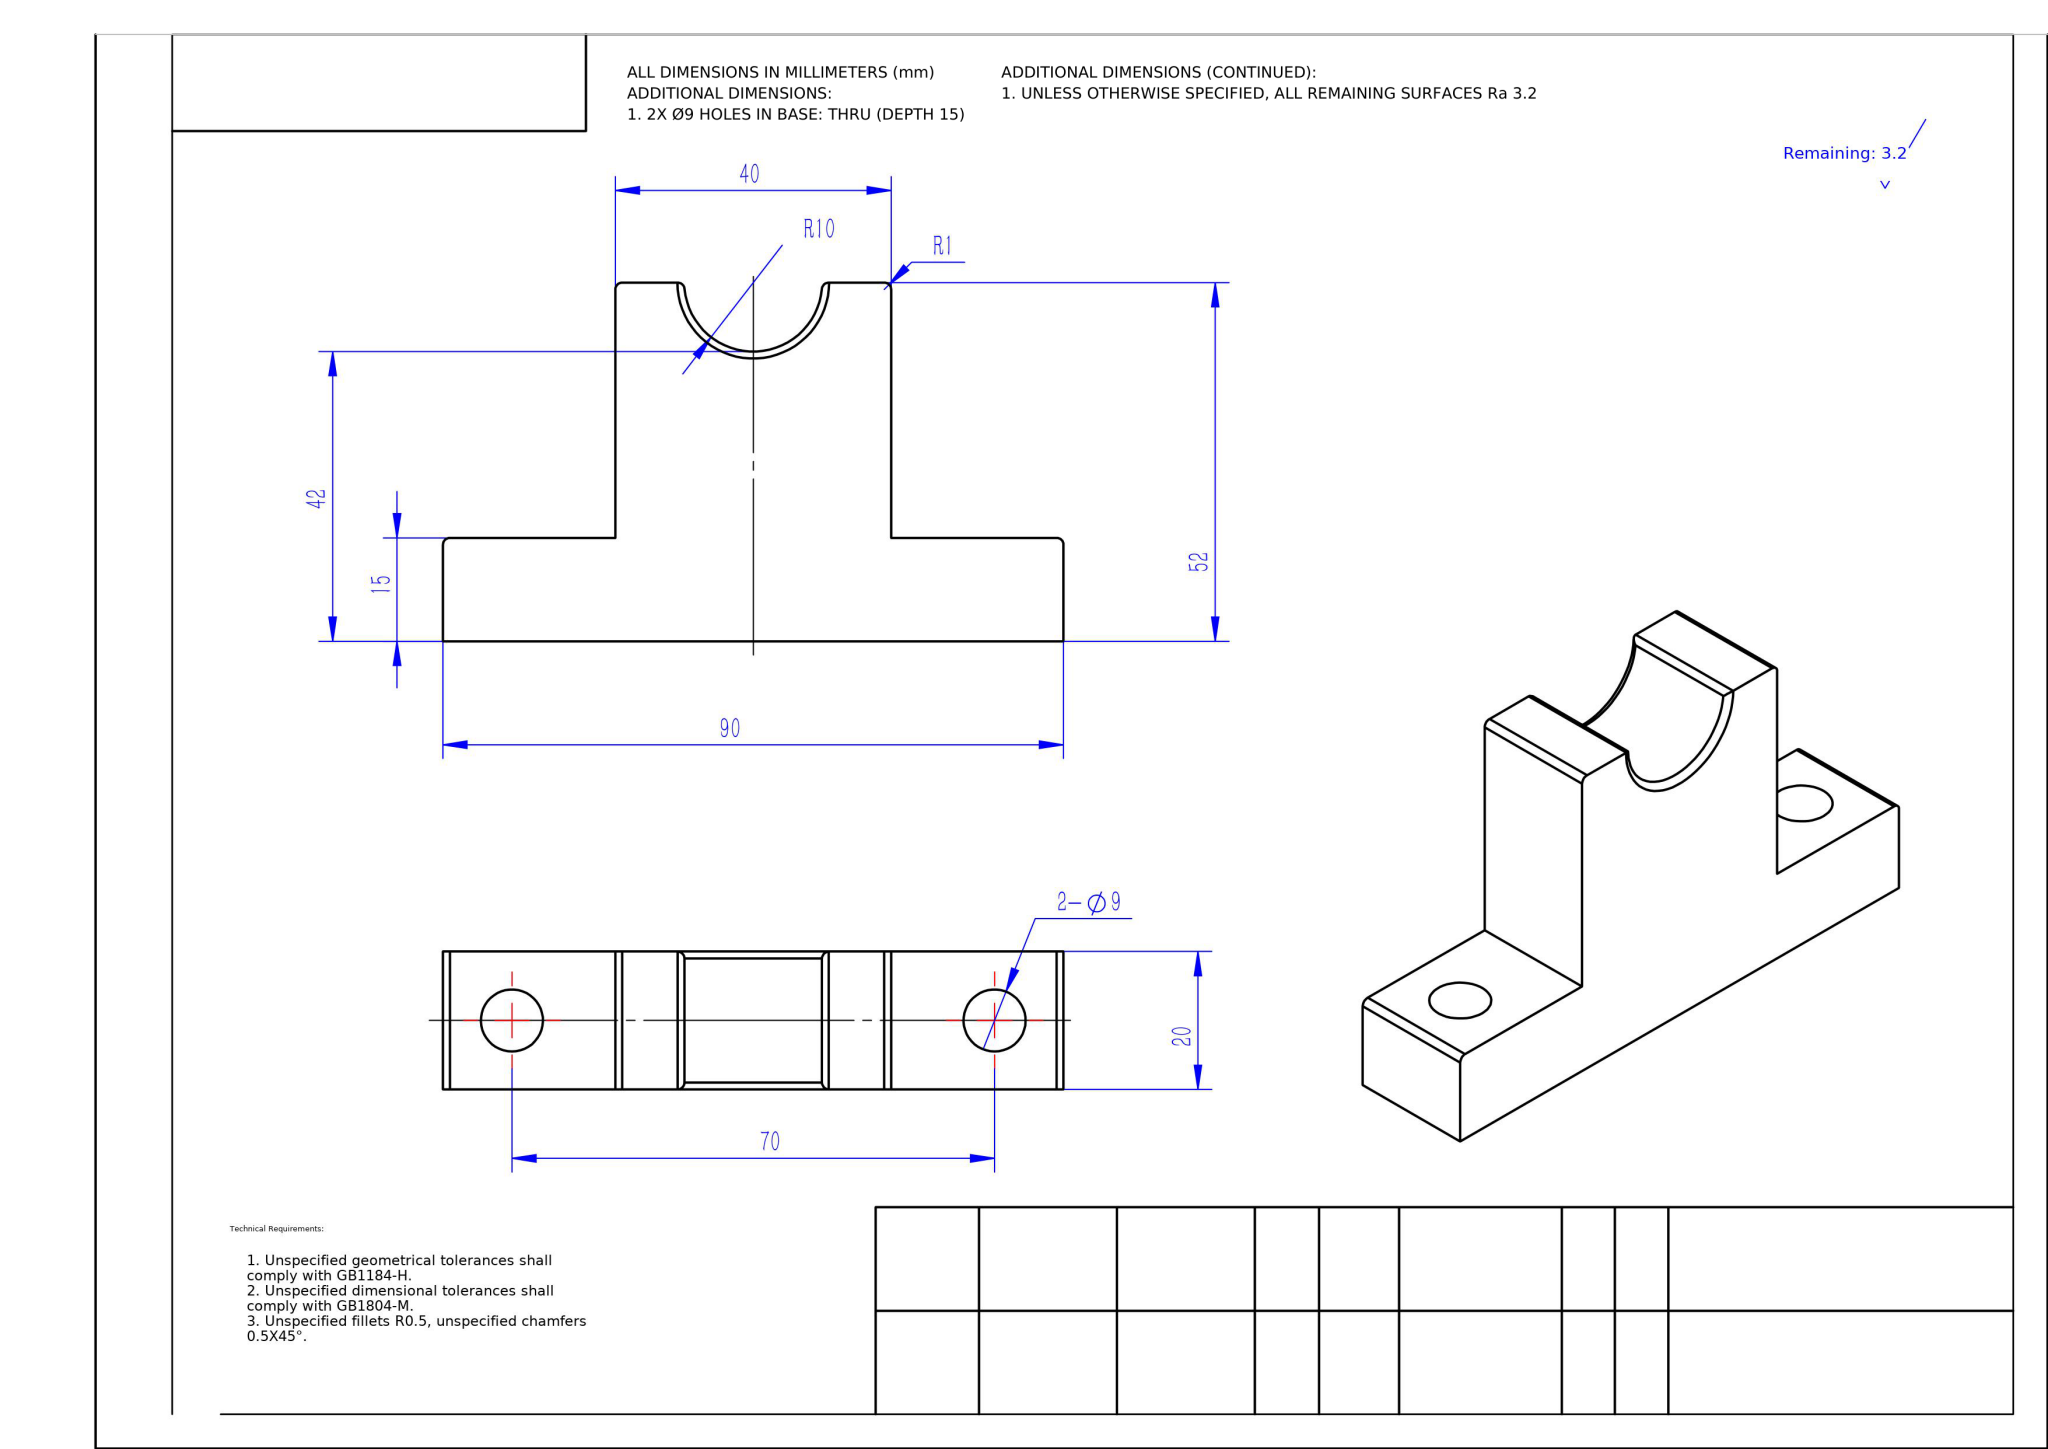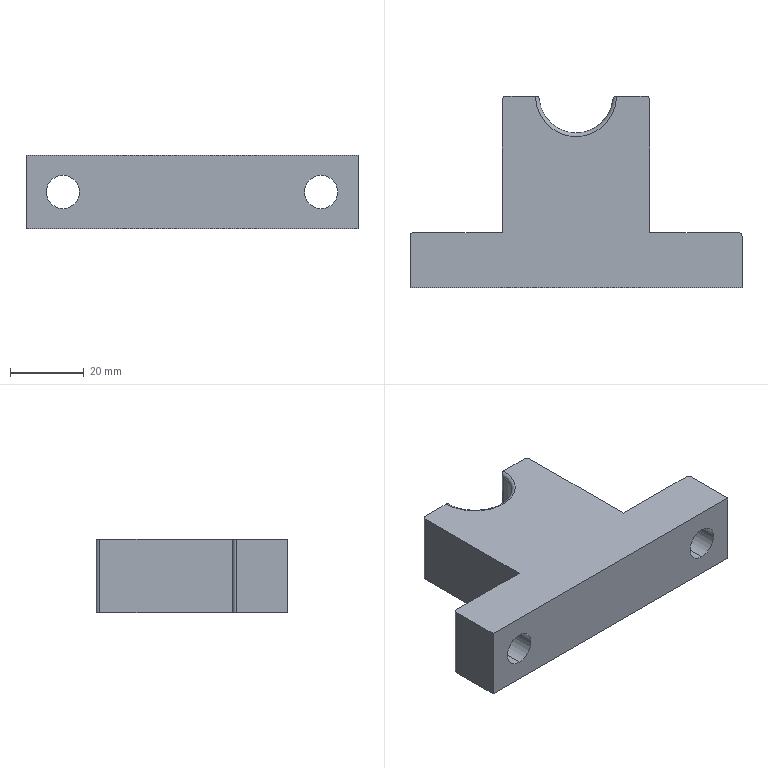Part | NX | mm | 1 solid | 24 faces | box 90 x 52 x 20 mm | volume 51512 mm3 | cylinder 11 | plane 11 | torus 2 | commonest cylinder face diameters 2 x6 9 x4 20 x1
STEP:
#1=COLOUR_RGB('',0.5294,0.549,0.549);
#2=FILL_AREA_STYLE_COLOUR('',#1);
#3=FILL_AREA_STYLE('',(#2));
#4=SURFACE_STYLE_FILL_AREA(#3);
#5=SURFACE_SIDE_STYLE('',(#4));
#6=SURFACE_STYLE_USAGE(.BOTH.,#5);
#7=PRESENTATION_STYLE_ASSIGNMENT((#6));
#8=CARTESIAN_POINT('',(-35.,0.,4.5));
#9=VERTEX_POINT('',#8);
#10=CARTESIAN_POINT('',(-35.,0.,-4.5));
#11=VERTEX_POINT('',#10);
#12=CARTESIAN_POINT('',(-35.,0.,0.));
#13=DIRECTION('',(0.,-1.,0.));
#14=DIRECTION('',(0.,0.,-1.));
#15=AXIS2_PLACEMENT_3D('',#12,#13,#14);
#16=CIRCLE('',#15,4.5);
#17=EDGE_CURVE('',#9,#11,#16,.T.);
#18=ORIENTED_EDGE('',*,*,#17,.T.);
#19=CARTESIAN_POINT('',(-35.,15.,-4.5));
#20=VERTEX_POINT('',#19);
#21=CARTESIAN_POINT('',(-35.,15.,-4.5));
#22=DIRECTION('',(0.,1.,0.));
#23=VECTOR('',#22,1000.);
#24=LINE('',#21,#23);
#25=EDGE_CURVE('',#11,#20,#24,.T.);
#26=ORIENTED_EDGE('',*,*,#25,.T.);
#27=CARTESIAN_POINT('',(-35.,15.,4.5));
#28=VERTEX_POINT('',#27);
#29=CARTESIAN_POINT('',(-35.,15.,0.));
#30=DIRECTION('',(0.,1.,0.));
#31=DIRECTION('',(0.,0.,1.));
#32=AXIS2_PLACEMENT_3D('',#29,#30,#31);
#33=CIRCLE('',#32,4.5);
#34=EDGE_CURVE('',#20,#28,#33,.T.);
#35=ORIENTED_EDGE('',*,*,#34,.T.);
#36=CARTESIAN_POINT('',(-35.,15.,4.5));
#37=DIRECTION('',(0.,1.,0.));
#38=VECTOR('',#37,1000.);
#39=LINE('',#36,#38);
#40=EDGE_CURVE('',#9,#28,#39,.T.);
#41=ORIENTED_EDGE('',*,*,#40,.F.);
#42=EDGE_LOOP('',(#18,#26,#35,#41));
#43=FACE_OUTER_BOUND('',#42,.T.);
#44=CARTESIAN_POINT('',(-35.,15.,0.));
#45=DIRECTION('',(0.,1.,0.));
#46=DIRECTION('',(0.,0.,1.));
#47=AXIS2_PLACEMENT_3D('',#44,#45,#46);
#48=CYLINDRICAL_SURFACE('',#47,4.5);
#49=ADVANCED_FACE('',(#43),#48,.F.);
#50=CARTESIAN_POINT('',(35.,0.,4.5));
#51=VERTEX_POINT('',#50);
#52=CARTESIAN_POINT('',(35.,0.,-4.5));
#53=VERTEX_POINT('',#52);
#54=CARTESIAN_POINT('',(35.,0.,0.));
#55=DIRECTION('',(0.,-1.,0.));
#56=DIRECTION('',(0.,0.,-1.));
#57=AXIS2_PLACEMENT_3D('',#54,#55,#56);
#58=CIRCLE('',#57,4.5);
#59=EDGE_CURVE('',#51,#53,#58,.T.);
#60=ORIENTED_EDGE('',*,*,#59,.T.);
#61=CARTESIAN_POINT('',(35.,15.,-4.5));
#62=VERTEX_POINT('',#61);
#63=CARTESIAN_POINT('',(35.,15.,-4.5));
#64=DIRECTION('',(0.,1.,0.));
#65=VECTOR('',#64,1000.);
#66=LINE('',#63,#65);
#67=EDGE_CURVE('',#53,#62,#66,.T.);
#68=ORIENTED_EDGE('',*,*,#67,.T.);
#69=CARTESIAN_POINT('',(35.,15.,4.5));
#70=VERTEX_POINT('',#69);
#71=CARTESIAN_POINT('',(35.,15.,0.));
#72=DIRECTION('',(0.,1.,0.));
#73=DIRECTION('',(0.,0.,1.));
#74=AXIS2_PLACEMENT_3D('',#71,#72,#73);
#75=CIRCLE('',#74,4.5);
#76=EDGE_CURVE('',#62,#70,#75,.T.);
#77=ORIENTED_EDGE('',*,*,#76,.T.);
#78=CARTESIAN_POINT('',(35.,15.,4.5));
#79=DIRECTION('',(0.,1.,0.));
#80=VECTOR('',#79,1000.);
#81=LINE('',#78,#80);
#82=EDGE_CURVE('',#51,#70,#81,.T.);
#83=ORIENTED_EDGE('',*,*,#82,.F.);
#84=EDGE_LOOP('',(#60,#68,#77,#83));
#85=FACE_OUTER_BOUND('',#84,.T.);
#86=CARTESIAN_POINT('',(35.,15.,0.));
#87=DIRECTION('',(0.,1.,0.));
#88=DIRECTION('',(0.,0.,1.));
#89=AXIS2_PLACEMENT_3D('',#86,#87,#88);
#90=CYLINDRICAL_SURFACE('',#89,4.5);
#91=ADVANCED_FACE('',(#85),#90,.F.);
#92=CARTESIAN_POINT('',(11.,52.,10.));
#93=VERTEX_POINT('',#92);
#94=CARTESIAN_POINT('',(19.,52.,10.));
#95=VERTEX_POINT('',#94);
#96=CARTESIAN_POINT('',(-45.,52.,10.));
#97=DIRECTION('',(1.,0.,0.));
#98=VECTOR('',#97,1000.);
#99=LINE('',#96,#98);
#100=EDGE_CURVE('',#93,#95,#99,.T.);
#101=ORIENTED_EDGE('',*,*,#100,.T.);
#102=CARTESIAN_POINT('',(19.,52.,-10.));
#103=VERTEX_POINT('',#102);
#104=CARTESIAN_POINT('',(19.,52.,-0.));
#105=DIRECTION('',(-0.,0.,-1.));
#106=VECTOR('',#105,1000.);
#107=LINE('',#104,#106);
#108=EDGE_CURVE('',#95,#103,#107,.T.);
#109=ORIENTED_EDGE('',*,*,#108,.T.);
#110=CARTESIAN_POINT('',(11.,52.,-10.));
#111=VERTEX_POINT('',#110);
#112=CARTESIAN_POINT('',(-45.,52.,-10.));
#113=DIRECTION('',(-1.,0.,0.));
#114=VECTOR('',#113,1000.);
#115=LINE('',#112,#114);
#116=EDGE_CURVE('',#103,#111,#115,.T.);
#117=ORIENTED_EDGE('',*,*,#116,.T.);
#118=CARTESIAN_POINT('',(10.954,52.,-9.999));
#119=VERTEX_POINT('',#118);
#120=CARTESIAN_POINT('',(11.,52.,-9.));
#121=DIRECTION('',(0.,1.,0.));
#122=DIRECTION('',(-0.,0.,-1.));
#123=AXIS2_PLACEMENT_3D('',#120,#121,#122);
#124=CIRCLE('',#123,1.);
#125=EDGE_CURVE('',#111,#119,#124,.T.);
#126=ORIENTED_EDGE('',*,*,#125,.T.);
#127=CARTESIAN_POINT('',(10.954,52.,9.999));
#128=VERTEX_POINT('',#127);
#129=CARTESIAN_POINT('',(10.954,52.,0.));
#130=DIRECTION('',(0.,0.,1.));
#131=VECTOR('',#130,1000.);
#132=LINE('',#129,#131);
#133=EDGE_CURVE('',#119,#128,#132,.T.);
#134=ORIENTED_EDGE('',*,*,#133,.T.);
#135=CARTESIAN_POINT('',(11.,52.,9.));
#136=DIRECTION('',(0.,1.,0.));
#137=DIRECTION('',(0.,0.,-1.));
#138=AXIS2_PLACEMENT_3D('',#135,#136,#137);
#139=CIRCLE('',#138,1.);
#140=EDGE_CURVE('',#128,#93,#139,.T.);
#141=ORIENTED_EDGE('',*,*,#140,.T.);
#142=EDGE_LOOP('',(#101,#109,#117,#126,#134,#141));
#143=FACE_OUTER_BOUND('',#142,.T.);
#144=CARTESIAN_POINT('',(0.,52.,0.));
#145=DIRECTION('',(0.,-1.,0.));
#146=DIRECTION('',(0.,0.,-1.));
#147=AXIS2_PLACEMENT_3D('',#144,#145,#146);
#148=PLANE('',#147);
#149=ADVANCED_FACE('',(#143),#148,.F.);
#150=CARTESIAN_POINT('',(45.,14.,-10.));
#151=VERTEX_POINT('',#150);
#152=CARTESIAN_POINT('',(45.,0.,-10.));
#153=VERTEX_POINT('',#152);
#154=CARTESIAN_POINT('',(45.,52.,-10.));
#155=DIRECTION('',(0.,-1.,0.));
#156=VECTOR('',#155,1000.);
#157=LINE('',#154,#156);
#158=EDGE_CURVE('',#151,#153,#157,.T.);
#159=ORIENTED_EDGE('',*,*,#158,.F.);
#160=CARTESIAN_POINT('',(45.,14.,10.));
#161=VERTEX_POINT('',#160);
#162=CARTESIAN_POINT('',(45.,14.,10.));
#163=DIRECTION('',(0.,0.,1.));
#164=VECTOR('',#163,1000.);
#165=LINE('',#162,#164);
#166=EDGE_CURVE('',#151,#161,#165,.T.);
#167=ORIENTED_EDGE('',*,*,#166,.T.);
#168=CARTESIAN_POINT('',(45.,0.,10.));
#169=VERTEX_POINT('',#168);
#170=CARTESIAN_POINT('',(45.,52.,10.));
#171=DIRECTION('',(0.,-1.,0.));
#172=VECTOR('',#171,1000.);
#173=LINE('',#170,#172);
#174=EDGE_CURVE('',#161,#169,#173,.T.);
#175=ORIENTED_EDGE('',*,*,#174,.T.);
#176=CARTESIAN_POINT('',(45.,0.,10.));
#177=DIRECTION('',(0.,0.,-1.));
#178=VECTOR('',#177,1000.);
#179=LINE('',#176,#178);
#180=EDGE_CURVE('',#169,#153,#179,.T.);
#181=ORIENTED_EDGE('',*,*,#180,.T.);
#182=EDGE_LOOP('',(#159,#167,#175,#181));
#183=FACE_OUTER_BOUND('',#182,.T.);
#184=CARTESIAN_POINT('',(45.,52.,10.));
#185=DIRECTION('',(-1.,0.,0.));
#186=DIRECTION('',(0.,0.,1.));
#187=AXIS2_PLACEMENT_3D('',#184,#185,#186);
#188=PLANE('',#187);
#189=ADVANCED_FACE('',(#183),#188,.F.);
#190=CARTESIAN_POINT('',(-45.,14.,10.));
#191=VERTEX_POINT('',#190);
#192=CARTESIAN_POINT('',(-45.,0.,10.));
#193=VERTEX_POINT('',#192);
#194=CARTESIAN_POINT('',(-45.,52.,10.));
#195=DIRECTION('',(0.,-1.,0.));
#196=VECTOR('',#195,1000.);
#197=LINE('',#194,#196);
#198=EDGE_CURVE('',#191,#193,#197,.T.);
#199=ORIENTED_EDGE('',*,*,#198,.F.);
#200=CARTESIAN_POINT('',(-45.,14.,-10.));
#201=VERTEX_POINT('',#200);
#202=CARTESIAN_POINT('',(-45.,14.,-10.));
#203=DIRECTION('',(0.,0.,-1.));
#204=VECTOR('',#203,1000.);
#205=LINE('',#202,#204);
#206=EDGE_CURVE('',#191,#201,#205,.T.);
#207=ORIENTED_EDGE('',*,*,#206,.T.);
#208=CARTESIAN_POINT('',(-45.,0.,-10.));
#209=VERTEX_POINT('',#208);
#210=CARTESIAN_POINT('',(-45.,52.,-10.));
#211=DIRECTION('',(0.,-1.,0.));
#212=VECTOR('',#211,1000.);
#213=LINE('',#210,#212);
#214=EDGE_CURVE('',#201,#209,#213,.T.);
#215=ORIENTED_EDGE('',*,*,#214,.T.);
#216=CARTESIAN_POINT('',(-45.,0.,10.));
#217=DIRECTION('',(0.,0.,1.));
#218=VECTOR('',#217,1000.);
#219=LINE('',#216,#218);
#220=EDGE_CURVE('',#209,#193,#219,.T.);
#221=ORIENTED_EDGE('',*,*,#220,.T.);
#222=EDGE_LOOP('',(#199,#207,#215,#221));
#223=FACE_OUTER_BOUND('',#222,.T.);
#224=CARTESIAN_POINT('',(-45.,52.,10.));
#225=DIRECTION('',(1.,0.,0.));
#226=DIRECTION('',(0.,0.,-1.));
#227=AXIS2_PLACEMENT_3D('',#224,#225,#226);
#228=PLANE('',#227);
#229=ADVANCED_FACE('',(#223),#228,.F.);
#230=CARTESIAN_POINT('',(-11.,52.,-10.));
#231=VERTEX_POINT('',#230);
#232=CARTESIAN_POINT('',(-19.,52.,-10.));
#233=VERTEX_POINT('',#232);
#234=CARTESIAN_POINT('',(-45.,52.,-10.));
#235=DIRECTION('',(-1.,0.,0.));
#236=VECTOR('',#235,1000.);
#237=LINE('',#234,#236);
#238=EDGE_CURVE('',#231,#233,#237,.T.);
#239=ORIENTED_EDGE('',*,*,#238,.F.);
#240=CARTESIAN_POINT('',(0.,52.,-10.));
#241=DIRECTION('',(0.,0.,1.));
#242=DIRECTION('',(1.,0.,0.));
#243=AXIS2_PLACEMENT_3D('',#240,#241,#242);
#244=CIRCLE('',#243,11.);
#245=EDGE_CURVE('',#231,#111,#244,.T.);
#246=ORIENTED_EDGE('',*,*,#245,.T.);
#247=ORIENTED_EDGE('',*,*,#116,.F.);
#248=CARTESIAN_POINT('',(20.,51.,-10.));
#249=VERTEX_POINT('',#248);
#250=CARTESIAN_POINT('',(19.,51.,-10.));
#251=DIRECTION('',(0.,0.,-1.));
#252=DIRECTION('',(1.,0.,0.));
#253=AXIS2_PLACEMENT_3D('',#250,#251,#252);
#254=CIRCLE('',#253,1.);
#255=EDGE_CURVE('',#103,#249,#254,.T.);
#256=ORIENTED_EDGE('',*,*,#255,.T.);
#257=CARTESIAN_POINT('',(20.,15.,-10.));
#258=VERTEX_POINT('',#257);
#259=CARTESIAN_POINT('',(20.,15.,-10.));
#260=DIRECTION('',(0.,1.,0.));
#261=VECTOR('',#260,1000.);
#262=LINE('',#259,#261);
#263=EDGE_CURVE('',#258,#249,#262,.T.);
#264=ORIENTED_EDGE('',*,*,#263,.F.);
#265=CARTESIAN_POINT('',(44.,15.,-10.));
#266=VERTEX_POINT('',#265);
#267=CARTESIAN_POINT('',(20.,15.,-10.));
#268=DIRECTION('',(-1.,0.,0.));
#269=VECTOR('',#268,1000.);
#270=LINE('',#267,#269);
#271=EDGE_CURVE('',#266,#258,#270,.T.);
#272=ORIENTED_EDGE('',*,*,#271,.F.);
#273=CARTESIAN_POINT('',(44.,14.,-10.));
#274=DIRECTION('',(0.,0.,-1.));
#275=DIRECTION('',(1.,-0.,0.));
#276=AXIS2_PLACEMENT_3D('',#273,#274,#275);
#277=CIRCLE('',#276,1.);
#278=EDGE_CURVE('',#266,#151,#277,.T.);
#279=ORIENTED_EDGE('',*,*,#278,.T.);
#280=ORIENTED_EDGE('',*,*,#158,.T.);
#281=CARTESIAN_POINT('',(-45.,0.,-10.));
#282=DIRECTION('',(-1.,0.,0.));
#283=VECTOR('',#282,1000.);
#284=LINE('',#281,#283);
#285=EDGE_CURVE('',#153,#209,#284,.T.);
#286=ORIENTED_EDGE('',*,*,#285,.T.);
#287=ORIENTED_EDGE('',*,*,#214,.F.);
#288=CARTESIAN_POINT('',(-44.,15.,-10.));
#289=VERTEX_POINT('',#288);
#290=CARTESIAN_POINT('',(-44.,14.,-10.));
#291=DIRECTION('',(0.,0.,-1.));
#292=DIRECTION('',(1.,0.,0.));
#293=AXIS2_PLACEMENT_3D('',#290,#291,#292);
#294=CIRCLE('',#293,1.);
#295=EDGE_CURVE('',#201,#289,#294,.T.);
#296=ORIENTED_EDGE('',*,*,#295,.T.);
#297=CARTESIAN_POINT('',(-20.,15.,-10.));
#298=VERTEX_POINT('',#297);
#299=CARTESIAN_POINT('',(-45.,15.,-10.));
#300=DIRECTION('',(-1.,0.,0.));
#301=VECTOR('',#300,1000.);
#302=LINE('',#299,#301);
#303=EDGE_CURVE('',#298,#289,#302,.T.);
#304=ORIENTED_EDGE('',*,*,#303,.F.);
#305=CARTESIAN_POINT('',(-20.,51.,-10.));
#306=VERTEX_POINT('',#305);
#307=CARTESIAN_POINT('',(-20.,15.,-10.));
#308=DIRECTION('',(0.,1.,0.));
#309=VECTOR('',#308,1000.);
#310=LINE('',#307,#309);
#311=EDGE_CURVE('',#298,#306,#310,.T.);
#312=ORIENTED_EDGE('',*,*,#311,.T.);
#313=CARTESIAN_POINT('',(-19.,51.,-10.));
#314=DIRECTION('',(0.,0.,-1.));
#315=DIRECTION('',(1.,0.,0.));
#316=AXIS2_PLACEMENT_3D('',#313,#314,#315);
#317=CIRCLE('',#316,1.);
#318=EDGE_CURVE('',#306,#233,#317,.T.);
#319=ORIENTED_EDGE('',*,*,#318,.T.);
#320=EDGE_LOOP('',(#239,#246,#247,#256,#264,#272,#279,#280,#286,#287,#296,#304,#312,#319));
#321=FACE_OUTER_BOUND('',#320,.T.);
#322=CARTESIAN_POINT('',(-45.,52.,-10.));
#323=DIRECTION('',(0.,0.,1.));
#324=DIRECTION('',(1.,0.,0.));
#325=AXIS2_PLACEMENT_3D('',#322,#323,#324);
#326=PLANE('',#325);
#327=ADVANCED_FACE('',(#321),#326,.F.);
#328=ORIENTED_EDGE('',*,*,#100,.F.);
#329=CARTESIAN_POINT('',(-11.,52.,10.));
#330=VERTEX_POINT('',#329);
#331=CARTESIAN_POINT('',(0.,52.,10.));
#332=DIRECTION('',(0.,0.,-1.));
#333=DIRECTION('',(-1.,0.,0.));
#334=AXIS2_PLACEMENT_3D('',#331,#332,#333);
#335=CIRCLE('',#334,11.);
#336=EDGE_CURVE('',#93,#330,#335,.T.);
#337=ORIENTED_EDGE('',*,*,#336,.T.);
#338=CARTESIAN_POINT('',(-19.,52.,10.));
#339=VERTEX_POINT('',#338);
#340=CARTESIAN_POINT('',(-45.,52.,10.));
#341=DIRECTION('',(1.,0.,0.));
#342=VECTOR('',#341,1000.);
#343=LINE('',#340,#342);
#344=EDGE_CURVE('',#339,#330,#343,.T.);
#345=ORIENTED_EDGE('',*,*,#344,.F.);
#346=CARTESIAN_POINT('',(-20.,51.,10.));
#347=VERTEX_POINT('',#346);
#348=CARTESIAN_POINT('',(-19.,51.,10.));
#349=DIRECTION('',(0.,0.,1.));
#350=DIRECTION('',(-1.,0.,0.));
#351=AXIS2_PLACEMENT_3D('',#348,#349,#350);
#352=CIRCLE('',#351,1.);
#353=EDGE_CURVE('',#339,#347,#352,.T.);
#354=ORIENTED_EDGE('',*,*,#353,.T.);
#355=CARTESIAN_POINT('',(-20.,15.,10.));
#356=VERTEX_POINT('',#355);
#357=CARTESIAN_POINT('',(-20.,15.,10.));
#358=DIRECTION('',(0.,1.,0.));
#359=VECTOR('',#358,1000.);
#360=LINE('',#357,#359);
#361=EDGE_CURVE('',#356,#347,#360,.T.);
#362=ORIENTED_EDGE('',*,*,#361,.F.);
#363=CARTESIAN_POINT('',(-44.,15.,10.));
#364=VERTEX_POINT('',#363);
#365=CARTESIAN_POINT('',(-45.,15.,10.));
#366=DIRECTION('',(1.,0.,0.));
#367=VECTOR('',#366,1000.);
#368=LINE('',#365,#367);
#369=EDGE_CURVE('',#364,#356,#368,.T.);
#370=ORIENTED_EDGE('',*,*,#369,.F.);
#371=CARTESIAN_POINT('',(-44.,14.,10.));
#372=DIRECTION('',(0.,0.,1.));
#373=DIRECTION('',(-1.,-0.,0.));
#374=AXIS2_PLACEMENT_3D('',#371,#372,#373);
#375=CIRCLE('',#374,1.);
#376=EDGE_CURVE('',#364,#191,#375,.T.);
#377=ORIENTED_EDGE('',*,*,#376,.T.);
#378=ORIENTED_EDGE('',*,*,#198,.T.);
#379=CARTESIAN_POINT('',(-45.,0.,10.));
#380=DIRECTION('',(1.,0.,0.));
#381=VECTOR('',#380,1000.);
#382=LINE('',#379,#381);
#383=EDGE_CURVE('',#193,#169,#382,.T.);
#384=ORIENTED_EDGE('',*,*,#383,.T.);
#385=ORIENTED_EDGE('',*,*,#174,.F.);
#386=CARTESIAN_POINT('',(44.,15.,10.));
#387=VERTEX_POINT('',#386);
#388=CARTESIAN_POINT('',(44.,14.,10.));
#389=DIRECTION('',(0.,0.,1.));
#390=DIRECTION('',(-1.,0.,0.));
#391=AXIS2_PLACEMENT_3D('',#388,#389,#390);
#392=CIRCLE('',#391,1.);
#393=EDGE_CURVE('',#161,#387,#392,.T.);
#394=ORIENTED_EDGE('',*,*,#393,.T.);
#395=CARTESIAN_POINT('',(20.,15.,10.));
#396=VERTEX_POINT('',#395);
#397=CARTESIAN_POINT('',(20.,15.,10.));
#398=DIRECTION('',(1.,0.,0.));
#399=VECTOR('',#398,1000.);
#400=LINE('',#397,#399);
#401=EDGE_CURVE('',#396,#387,#400,.T.);
#402=ORIENTED_EDGE('',*,*,#401,.F.);
#403=CARTESIAN_POINT('',(20.,51.,10.));
#404=VERTEX_POINT('',#403);
#405=CARTESIAN_POINT('',(20.,15.,10.));
#406=DIRECTION('',(0.,1.,0.));
#407=VECTOR('',#406,1000.);
#408=LINE('',#405,#407);
#409=EDGE_CURVE('',#396,#404,#408,.T.);
#410=ORIENTED_EDGE('',*,*,#409,.T.);
#411=CARTESIAN_POINT('',(19.,51.,10.));
#412=DIRECTION('',(0.,0.,1.));
#413=DIRECTION('',(-1.,0.,0.));
#414=AXIS2_PLACEMENT_3D('',#411,#412,#413);
#415=CIRCLE('',#414,1.);
#416=EDGE_CURVE('',#404,#95,#415,.T.);
#417=ORIENTED_EDGE('',*,*,#416,.T.);
#418=EDGE_LOOP('',(#328,#337,#345,#354,#362,#370,#377,#378,#384,#385,#394,#402,#410,#417));
#419=FACE_OUTER_BOUND('',#418,.T.);
#420=CARTESIAN_POINT('',(-45.,52.,10.));
#421=DIRECTION('',(0.,0.,-1.));
#422=DIRECTION('',(-1.,0.,0.));
#423=AXIS2_PLACEMENT_3D('',#420,#421,#422);
#424=PLANE('',#423);
#425=ADVANCED_FACE('',(#419),#424,.F.);
#426=ORIENTED_EDGE('',*,*,#238,.T.);
#427=CARTESIAN_POINT('',(-19.,52.,0.));
#428=DIRECTION('',(0.,0.,1.));
#429=VECTOR('',#428,1000.);
#430=LINE('',#427,#429);
#431=EDGE_CURVE('',#233,#339,#430,.T.);
#432=ORIENTED_EDGE('',*,*,#431,.T.);
#433=ORIENTED_EDGE('',*,*,#344,.T.);
#434=CARTESIAN_POINT('',(-10.954,52.,9.999));
#435=VERTEX_POINT('',#434);
#436=CARTESIAN_POINT('',(-11.,52.,9.));
#437=DIRECTION('',(0.,1.,0.));
#438=DIRECTION('',(0.,0.,-1.));
#439=AXIS2_PLACEMENT_3D('',#436,#437,#438);
#440=CIRCLE('',#439,1.);
#441=EDGE_CURVE('',#330,#435,#440,.T.);
#442=ORIENTED_EDGE('',*,*,#441,.T.);
#443=CARTESIAN_POINT('',(-10.954,52.,-9.999));
#444=VERTEX_POINT('',#443);
#445=CARTESIAN_POINT('',(-10.954,52.,0.));
#446=DIRECTION('',(0.,0.,-1.));
#447=VECTOR('',#446,1000.);
#448=LINE('',#445,#447);
#449=EDGE_CURVE('',#435,#444,#448,.T.);
#450=ORIENTED_EDGE('',*,*,#449,.T.);
#451=CARTESIAN_POINT('',(-11.,52.,-9.));
#452=DIRECTION('',(0.,1.,0.));
#453=DIRECTION('',(0.,0.,-1.));
#454=AXIS2_PLACEMENT_3D('',#451,#452,#453);
#455=CIRCLE('',#454,1.);
#456=EDGE_CURVE('',#444,#231,#455,.T.);
#457=ORIENTED_EDGE('',*,*,#456,.T.);
#458=EDGE_LOOP('',(#426,#432,#433,#442,#450,#457));
#459=FACE_OUTER_BOUND('',#458,.T.);
#460=CARTESIAN_POINT('',(0.,52.,0.));
#461=DIRECTION('',(0.,-1.,0.));
#462=DIRECTION('',(0.,0.,-1.));
#463=AXIS2_PLACEMENT_3D('',#460,#461,#462);
#464=PLANE('',#463);
#465=ADVANCED_FACE('',(#459),#464,.F.);
#466=ORIENTED_EDGE('',*,*,#17,.F.);
#467=CARTESIAN_POINT('',(-35.,0.,0.));
#468=DIRECTION('',(0.,-1.,0.));
#469=DIRECTION('',(0.,0.,-1.));
#470=AXIS2_PLACEMENT_3D('',#467,#468,#469);
#471=CIRCLE('',#470,4.5);
#472=EDGE_CURVE('',#11,#9,#471,.T.);
#473=ORIENTED_EDGE('',*,*,#472,.F.);
#474=EDGE_LOOP('',(#466,#473));
#475=FACE_BOUND('',#474,.T.);
#476=ORIENTED_EDGE('',*,*,#59,.F.);
#477=CARTESIAN_POINT('',(35.,0.,0.));
#478=DIRECTION('',(0.,-1.,0.));
#479=DIRECTION('',(0.,0.,-1.));
#480=AXIS2_PLACEMENT_3D('',#477,#478,#479);
#481=CIRCLE('',#480,4.5);
#482=EDGE_CURVE('',#53,#51,#481,.T.);
#483=ORIENTED_EDGE('',*,*,#482,.F.);
#484=EDGE_LOOP('',(#476,#483));
#485=FACE_BOUND('',#484,.T.);
#486=ORIENTED_EDGE('',*,*,#180,.F.);
#487=ORIENTED_EDGE('',*,*,#383,.F.);
#488=ORIENTED_EDGE('',*,*,#220,.F.);
#489=ORIENTED_EDGE('',*,*,#285,.F.);
#490=EDGE_LOOP('',(#486,#487,#488,#489));
#491=FACE_OUTER_BOUND('',#490,.T.);
#492=CARTESIAN_POINT('',(0.,0.,0.));
#493=DIRECTION('',(0.,-1.,0.));
#494=DIRECTION('',(0.,0.,-1.));
#495=AXIS2_PLACEMENT_3D('',#492,#493,#494);
#496=PLANE('',#495);
#497=ADVANCED_FACE('',(#475,#485,#491),#496,.T.);
#498=ORIENTED_EDGE('',*,*,#263,.T.);
#499=CARTESIAN_POINT('',(20.,51.,-10.));
#500=DIRECTION('',(0.,0.,1.));
#501=VECTOR('',#500,1000.);
#502=LINE('',#499,#501);
#503=EDGE_CURVE('',#249,#404,#502,.T.);
#504=ORIENTED_EDGE('',*,*,#503,.T.);
#505=ORIENTED_EDGE('',*,*,#409,.F.);
#506=CARTESIAN_POINT('',(20.,15.,-10.));
#507=DIRECTION('',(0.,0.,1.));
#508=VECTOR('',#507,1000.);
#509=LINE('',#506,#508);
#510=EDGE_CURVE('',#258,#396,#509,.T.);
#511=ORIENTED_EDGE('',*,*,#510,.F.);
#512=EDGE_LOOP('',(#498,#504,#505,#511));
#513=FACE_OUTER_BOUND('',#512,.T.);
#514=CARTESIAN_POINT('',(20.,15.,-10.));
#515=DIRECTION('',(-1.,0.,0.));
#516=DIRECTION('',(0.,0.,1.));
#517=AXIS2_PLACEMENT_3D('',#514,#515,#516);
#518=PLANE('',#517);
#519=ADVANCED_FACE('',(#513),#518,.F.);
#520=CARTESIAN_POINT('',(35.,15.,0.));
#521=DIRECTION('',(0.,1.,0.));
#522=DIRECTION('',(0.,0.,1.));
#523=AXIS2_PLACEMENT_3D('',#520,#521,#522);
#524=CIRCLE('',#523,4.5);
#525=EDGE_CURVE('',#70,#62,#524,.T.);
#526=ORIENTED_EDGE('',*,*,#525,.F.);
#527=ORIENTED_EDGE('',*,*,#76,.F.);
#528=EDGE_LOOP('',(#526,#527));
#529=FACE_BOUND('',#528,.T.);
#530=ORIENTED_EDGE('',*,*,#401,.T.);
#531=CARTESIAN_POINT('',(44.,15.,-10.));
#532=DIRECTION('',(0.,0.,-1.));
#533=VECTOR('',#532,1000.);
#534=LINE('',#531,#533);
#535=EDGE_CURVE('',#387,#266,#534,.T.);
#536=ORIENTED_EDGE('',*,*,#535,.T.);
#537=ORIENTED_EDGE('',*,*,#271,.T.);
#538=ORIENTED_EDGE('',*,*,#510,.T.);
#539=EDGE_LOOP('',(#530,#536,#537,#538));
#540=FACE_OUTER_BOUND('',#539,.T.);
#541=CARTESIAN_POINT('',(0.,15.,0.));
#542=DIRECTION('',(0.,1.,0.));
#543=DIRECTION('',(0.,0.,1.));
#544=AXIS2_PLACEMENT_3D('',#541,#542,#543);
#545=PLANE('',#544);
#546=ADVANCED_FACE('',(#529,#540),#545,.T.);
#547=ORIENTED_EDGE('',*,*,#361,.T.);
#548=CARTESIAN_POINT('',(-20.,51.,-10.));
#549=DIRECTION('',(-0.,0.,-1.));
#550=VECTOR('',#549,1000.);
#551=LINE('',#548,#550);
#552=EDGE_CURVE('',#347,#306,#551,.T.);
#553=ORIENTED_EDGE('',*,*,#552,.T.);
#554=ORIENTED_EDGE('',*,*,#311,.F.);
#555=CARTESIAN_POINT('',(-20.,15.,-10.));
#556=DIRECTION('',(-0.,0.,-1.));
#557=VECTOR('',#556,1000.);
#558=LINE('',#555,#557);
#559=EDGE_CURVE('',#356,#298,#558,.T.);
#560=ORIENTED_EDGE('',*,*,#559,.F.);
#561=EDGE_LOOP('',(#547,#553,#554,#560));
#562=FACE_OUTER_BOUND('',#561,.T.);
#563=CARTESIAN_POINT('',(-20.,15.,-10.));
#564=DIRECTION('',(1.,0.,-0.));
#565=DIRECTION('',(-0.,0.,-1.));
#566=AXIS2_PLACEMENT_3D('',#563,#564,#565);
#567=PLANE('',#566);
#568=ADVANCED_FACE('',(#562),#567,.F.);
#569=CARTESIAN_POINT('',(-35.,15.,0.));
#570=DIRECTION('',(0.,1.,0.));
#571=DIRECTION('',(0.,0.,1.));
#572=AXIS2_PLACEMENT_3D('',#569,#570,#571);
#573=CIRCLE('',#572,4.5);
#574=EDGE_CURVE('',#28,#20,#573,.T.);
#575=ORIENTED_EDGE('',*,*,#574,.F.);
#576=ORIENTED_EDGE('',*,*,#34,.F.);
#577=EDGE_LOOP('',(#575,#576));
#578=FACE_BOUND('',#577,.T.);
#579=ORIENTED_EDGE('',*,*,#303,.T.);
#580=CARTESIAN_POINT('',(-44.,15.,10.));
#581=DIRECTION('',(0.,0.,1.));
#582=VECTOR('',#581,1000.);
#583=LINE('',#580,#582);
#584=EDGE_CURVE('',#289,#364,#583,.T.);
#585=ORIENTED_EDGE('',*,*,#584,.T.);
#586=ORIENTED_EDGE('',*,*,#369,.T.);
#587=ORIENTED_EDGE('',*,*,#559,.T.);
#588=EDGE_LOOP('',(#579,#585,#586,#587));
#589=FACE_OUTER_BOUND('',#588,.T.);
#590=CARTESIAN_POINT('',(0.,15.,0.));
#591=DIRECTION('',(0.,1.,0.));
#592=DIRECTION('',(0.,0.,1.));
#593=AXIS2_PLACEMENT_3D('',#590,#591,#592);
#594=PLANE('',#593);
#595=ADVANCED_FACE('',(#578,#589),#594,.T.);
#596=CARTESIAN_POINT('',(-9.959,51.091,9.));
#597=VERTEX_POINT('',#596);
#598=CARTESIAN_POINT('',(9.959,51.091,9.));
#599=VERTEX_POINT('',#598);
#600=CARTESIAN_POINT('',(0.,52.,9.));
#601=DIRECTION('',(0.,0.,1.));
#602=DIRECTION('',(-1.,0.,0.));
#603=AXIS2_PLACEMENT_3D('',#600,#601,#602);
#604=CIRCLE('',#603,10.);
#605=EDGE_CURVE('',#597,#599,#604,.T.);
#606=ORIENTED_EDGE('',*,*,#605,.T.);
#607=CARTESIAN_POINT('',(9.959,51.091,-9.));
#608=VERTEX_POINT('',#607);
#609=CARTESIAN_POINT('',(9.959,51.091,-10.001));
#610=DIRECTION('',(0.,0.,-1.));
#611=VECTOR('',#610,1000.);
#612=LINE('',#609,#611);
#613=EDGE_CURVE('',#599,#608,#612,.T.);
#614=ORIENTED_EDGE('',*,*,#613,.T.);
#615=CARTESIAN_POINT('',(-9.959,51.091,-9.));
#616=VERTEX_POINT('',#615);
#617=CARTESIAN_POINT('',(0.,52.,-9.));
#618=DIRECTION('',(0.,0.,-1.));
#619=DIRECTION('',(1.,0.,0.));
#620=AXIS2_PLACEMENT_3D('',#617,#618,#619);
#621=CIRCLE('',#620,10.);
#622=EDGE_CURVE('',#608,#616,#621,.T.);
#623=ORIENTED_EDGE('',*,*,#622,.T.);
#624=CARTESIAN_POINT('',(-9.959,51.091,-10.001));
#625=DIRECTION('',(0.,0.,1.));
#626=VECTOR('',#625,1000.);
#627=LINE('',#624,#626);
#628=EDGE_CURVE('',#616,#597,#627,.T.);
#629=ORIENTED_EDGE('',*,*,#628,.T.);
#630=EDGE_LOOP('',(#606,#614,#623,#629));
#631=FACE_OUTER_BOUND('',#630,.T.);
#632=CARTESIAN_POINT('',(0.,52.,-10.001));
#633=DIRECTION('',(0.,0.,1.));
#634=DIRECTION('',(1.,0.,0.));
#635=AXIS2_PLACEMENT_3D('',#632,#633,#634);
#636=CYLINDRICAL_SURFACE('',#635,10.);
#637=ADVANCED_FACE('',(#631),#636,.F.);
#638=ORIENTED_EDGE('',*,*,#67,.F.);
#639=ORIENTED_EDGE('',*,*,#482,.T.);
#640=ORIENTED_EDGE('',*,*,#82,.T.);
#641=ORIENTED_EDGE('',*,*,#525,.T.);
#642=EDGE_LOOP('',(#638,#639,#640,#641));
#643=FACE_OUTER_BOUND('',#642,.T.);
#644=CARTESIAN_POINT('',(35.,15.,0.));
#645=DIRECTION('',(0.,1.,0.));
#646=DIRECTION('',(0.,0.,1.));
#647=AXIS2_PLACEMENT_3D('',#644,#645,#646);
#648=CYLINDRICAL_SURFACE('',#647,4.5);
#649=ADVANCED_FACE('',(#643),#648,.F.);
#650=ORIENTED_EDGE('',*,*,#25,.F.);
#651=ORIENTED_EDGE('',*,*,#472,.T.);
#652=ORIENTED_EDGE('',*,*,#40,.T.);
#653=ORIENTED_EDGE('',*,*,#574,.T.);
#654=EDGE_LOOP('',(#650,#651,#652,#653));
#655=FACE_OUTER_BOUND('',#654,.T.);
#656=CARTESIAN_POINT('',(-35.,15.,0.));
#657=DIRECTION('',(0.,1.,0.));
#658=DIRECTION('',(0.,0.,1.));
#659=AXIS2_PLACEMENT_3D('',#656,#657,#658);
#660=CYLINDRICAL_SURFACE('',#659,4.5);
#661=ADVANCED_FACE('',(#655),#660,.F.);
#662=ORIENTED_EDGE('',*,*,#336,.F.);
#663=ORIENTED_EDGE('',*,*,#140,.F.);
#664=CARTESIAN_POINT('',(9.959,51.091,9.));
#665=CARTESIAN_POINT('',(9.968,51.196,9.11));
#666=CARTESIAN_POINT('',(9.994,51.3,9.222));
#667=CARTESIAN_POINT('',(10.081,51.498,9.435));
#668=CARTESIAN_POINT('',(10.14,51.593,9.538));
#669=CARTESIAN_POINT('',(10.262,51.724,9.682));
#670=CARTESIAN_POINT('',(10.307,51.765,9.727));
#671=CARTESIAN_POINT('',(10.409,51.841,9.81));
#672=CARTESIAN_POINT('',(10.466,51.876,9.849));
#673=CARTESIAN_POINT('',(10.653,51.963,9.948));
#674=CARTESIAN_POINT('',(10.8,52.,9.992));
#675=CARTESIAN_POINT('',(10.954,52.,9.999));
#676=B_SPLINE_CURVE_WITH_KNOTS('',3,(#664,#665,#666,#667,#668,#669,#670,#671,#672,#673,#674,#675),.UNSPECIFIED.,.F.,.F.,(4,2,2,2,2,4),(-0.00000632,0.0004515,0.0009093,0.001138,0.001367,0.001825),.UNSPECIFIED.);
#677=EDGE_CURVE('',#599,#128,#676,.T.);
#678=ORIENTED_EDGE('',*,*,#677,.F.);
#679=ORIENTED_EDGE('',*,*,#605,.F.);
#680=CARTESIAN_POINT('',(-10.954,52.,9.999));
#681=CARTESIAN_POINT('',(-10.8,52.,9.992));
#682=CARTESIAN_POINT('',(-10.653,51.963,9.948));
#683=CARTESIAN_POINT('',(-10.466,51.876,9.849));
#684=CARTESIAN_POINT('',(-10.409,51.841,9.81));
#685=CARTESIAN_POINT('',(-10.307,51.765,9.727));
#686=CARTESIAN_POINT('',(-10.262,51.724,9.682));
#687=CARTESIAN_POINT('',(-10.14,51.593,9.538));
#688=CARTESIAN_POINT('',(-10.081,51.498,9.435));
#689=CARTESIAN_POINT('',(-9.994,51.3,9.222));
#690=CARTESIAN_POINT('',(-9.968,51.195,9.11));
#691=CARTESIAN_POINT('',(-9.959,51.091,9.));
#692=B_SPLINE_CURVE_WITH_KNOTS('',3,(#680,#681,#682,#683,#684,#685,#686,#687,#688,#689,#690,#691),.UNSPECIFIED.,.F.,.F.,(4,2,2,2,2,4),(0.,0.0004553,0.000683,0.0009107,0.001366,0.001821),.UNSPECIFIED.);
#693=EDGE_CURVE('',#435,#597,#692,.T.);
#694=ORIENTED_EDGE('',*,*,#693,.F.);
#695=ORIENTED_EDGE('',*,*,#441,.F.);
#696=EDGE_LOOP('',(#662,#663,#678,#679,#694,#695));
#697=FACE_OUTER_BOUND('',#696,.T.);
#698=CARTESIAN_POINT('',(0.,52.,9.));
#699=DIRECTION('',(0.,0.,-1.));
#700=DIRECTION('',(-1.,0.,0.));
#701=AXIS2_PLACEMENT_3D('',#698,#699,#700);
#702=TOROIDAL_SURFACE('',#701,11.,1.);
#703=ADVANCED_FACE('',(#697),#702,.T.);
#704=ORIENTED_EDGE('',*,*,#677,.T.);
#705=ORIENTED_EDGE('',*,*,#133,.F.);
#706=CARTESIAN_POINT('',(9.959,51.091,-9.));
#707=CARTESIAN_POINT('',(9.968,51.196,-9.11));
#708=CARTESIAN_POINT('',(9.994,51.3,-9.222));
#709=CARTESIAN_POINT('',(10.081,51.498,-9.435));
#710=CARTESIAN_POINT('',(10.14,51.593,-9.538));
#711=CARTESIAN_POINT('',(10.262,51.724,-9.682));
#712=CARTESIAN_POINT('',(10.307,51.765,-9.727));
#713=CARTESIAN_POINT('',(10.409,51.841,-9.81));
#714=CARTESIAN_POINT('',(10.466,51.876,-9.849));
#715=CARTESIAN_POINT('',(10.653,51.963,-9.948));
#716=CARTESIAN_POINT('',(10.8,52.,-9.992));
#717=CARTESIAN_POINT('',(10.954,52.,-9.999));
#718=B_SPLINE_CURVE_WITH_KNOTS('',3,(#706,#707,#708,#709,#710,#711,#712,#713,#714,#715,#716,#717),.UNSPECIFIED.,.F.,.F.,(4,2,2,2,2,4),(-0.00000632,0.0004515,0.0009093,0.001138,0.001367,0.001825),.UNSPECIFIED.);
#719=EDGE_CURVE('',#608,#119,#718,.T.);
#720=ORIENTED_EDGE('',*,*,#719,.F.);
#721=ORIENTED_EDGE('',*,*,#613,.F.);
#722=EDGE_LOOP('',(#704,#705,#720,#721));
#723=FACE_OUTER_BOUND('',#722,.T.);
#724=CARTESIAN_POINT('',(10.954,51.,-10.001));
#725=DIRECTION('',(0.,0.,1.));
#726=DIRECTION('',(1.,0.,0.));
#727=AXIS2_PLACEMENT_3D('',#724,#725,#726);
#728=CYLINDRICAL_SURFACE('',#727,1.);
#729=ADVANCED_FACE('',(#723),#728,.T.);
#730=ORIENTED_EDGE('',*,*,#693,.T.);
#731=ORIENTED_EDGE('',*,*,#628,.F.);
#732=CARTESIAN_POINT('',(-10.954,52.,-9.999));
#733=CARTESIAN_POINT('',(-10.8,52.,-9.992));
#734=CARTESIAN_POINT('',(-10.653,51.963,-9.948));
#735=CARTESIAN_POINT('',(-10.466,51.876,-9.849));
#736=CARTESIAN_POINT('',(-10.409,51.841,-9.81));
#737=CARTESIAN_POINT('',(-10.307,51.765,-9.727));
#738=CARTESIAN_POINT('',(-10.262,51.724,-9.682));
#739=CARTESIAN_POINT('',(-10.14,51.593,-9.538));
#740=CARTESIAN_POINT('',(-10.081,51.498,-9.435));
#741=CARTESIAN_POINT('',(-9.994,51.3,-9.222));
#742=CARTESIAN_POINT('',(-9.968,51.195,-9.11));
#743=CARTESIAN_POINT('',(-9.959,51.091,-9.));
#744=B_SPLINE_CURVE_WITH_KNOTS('',3,(#732,#733,#734,#735,#736,#737,#738,#739,#740,#741,#742,#743),.UNSPECIFIED.,.F.,.F.,(4,2,2,2,2,4),(0.,0.0004553,0.000683,0.0009107,0.001366,0.001821),.UNSPECIFIED.);
#745=EDGE_CURVE('',#444,#616,#744,.T.);
#746=ORIENTED_EDGE('',*,*,#745,.F.);
#747=ORIENTED_EDGE('',*,*,#449,.F.);
#748=EDGE_LOOP('',(#730,#731,#746,#747));
#749=FACE_OUTER_BOUND('',#748,.T.);
#750=CARTESIAN_POINT('',(-10.954,51.,-10.001));
#751=DIRECTION('',(0.,0.,1.));
#752=DIRECTION('',(1.,0.,0.));
#753=AXIS2_PLACEMENT_3D('',#750,#751,#752);
#754=CYLINDRICAL_SURFACE('',#753,1.);
#755=ADVANCED_FACE('',(#749),#754,.T.);
#756=ORIENTED_EDGE('',*,*,#125,.F.);
#757=ORIENTED_EDGE('',*,*,#245,.F.);
#758=ORIENTED_EDGE('',*,*,#456,.F.);
#759=ORIENTED_EDGE('',*,*,#745,.T.);
#760=ORIENTED_EDGE('',*,*,#622,.F.);
#761=ORIENTED_EDGE('',*,*,#719,.T.);
#762=EDGE_LOOP('',(#756,#757,#758,#759,#760,#761));
#763=FACE_OUTER_BOUND('',#762,.T.);
#764=CARTESIAN_POINT('',(0.,52.,-9.));
#765=DIRECTION('',(0.,0.,1.));
#766=DIRECTION('',(1.,0.,0.));
#767=AXIS2_PLACEMENT_3D('',#764,#765,#766);
#768=TOROIDAL_SURFACE('',#767,11.,1.);
#769=ADVANCED_FACE('',(#763),#768,.T.);
#770=ORIENTED_EDGE('',*,*,#393,.F.);
#771=ORIENTED_EDGE('',*,*,#166,.F.);
#772=ORIENTED_EDGE('',*,*,#278,.F.);
#773=ORIENTED_EDGE('',*,*,#535,.F.);
#774=EDGE_LOOP('',(#770,#771,#772,#773));
#775=FACE_OUTER_BOUND('',#774,.T.);
#776=CARTESIAN_POINT('',(44.,14.,0.));
#777=DIRECTION('',(0.,0.,1.));
#778=DIRECTION('',(1.,0.,0.));
#779=AXIS2_PLACEMENT_3D('',#776,#777,#778);
#780=CYLINDRICAL_SURFACE('',#779,1.);
#781=ADVANCED_FACE('',(#775),#780,.T.);
#782=ORIENTED_EDGE('',*,*,#295,.F.);
#783=ORIENTED_EDGE('',*,*,#206,.F.);
#784=ORIENTED_EDGE('',*,*,#376,.F.);
#785=ORIENTED_EDGE('',*,*,#584,.F.);
#786=EDGE_LOOP('',(#782,#783,#784,#785));
#787=FACE_OUTER_BOUND('',#786,.T.);
#788=CARTESIAN_POINT('',(-44.,14.,0.));
#789=DIRECTION('',(0.,0.,-1.));
#790=DIRECTION('',(-1.,0.,0.));
#791=AXIS2_PLACEMENT_3D('',#788,#789,#790);
#792=CYLINDRICAL_SURFACE('',#791,1.);
#793=ADVANCED_FACE('',(#787),#792,.T.);
#794=ORIENTED_EDGE('',*,*,#255,.F.);
#795=ORIENTED_EDGE('',*,*,#108,.F.);
#796=ORIENTED_EDGE('',*,*,#416,.F.);
#797=ORIENTED_EDGE('',*,*,#503,.F.);
#798=EDGE_LOOP('',(#794,#795,#796,#797));
#799=FACE_OUTER_BOUND('',#798,.T.);
#800=CARTESIAN_POINT('',(19.,51.,-10.));
#801=DIRECTION('',(0.,0.,1.));
#802=DIRECTION('',(1.,0.,0.));
#803=AXIS2_PLACEMENT_3D('',#800,#801,#802);
#804=CYLINDRICAL_SURFACE('',#803,1.);
#805=ADVANCED_FACE('',(#799),#804,.T.);
#806=ORIENTED_EDGE('',*,*,#353,.F.);
#807=ORIENTED_EDGE('',*,*,#431,.F.);
#808=ORIENTED_EDGE('',*,*,#318,.F.);
#809=ORIENTED_EDGE('',*,*,#552,.F.);
#810=EDGE_LOOP('',(#806,#807,#808,#809));
#811=FACE_OUTER_BOUND('',#810,.T.);
#812=CARTESIAN_POINT('',(-19.,51.,-10.));
#813=DIRECTION('',(-0.,0.,-1.));
#814=DIRECTION('',(-1.,0.,0.));
#815=AXIS2_PLACEMENT_3D('',#812,#813,#814);
#816=CYLINDRICAL_SURFACE('',#815,1.);
#817=ADVANCED_FACE('',(#811),#816,.T.);
#818=CLOSED_SHELL('',(#49,#91,#149,#189,#229,#327,#425,#465,#497,#519,#546,#568,#595,#637,#649,#661,#703,#729,#755,#769,#781,#793,#805,#817));
#819=MANIFOLD_SOLID_BREP('',#818);
#820=CARTESIAN_POINT('',(0.,0.,0.));
#821=DIRECTION('',(0.,0.,1.));
#822=DIRECTION('',(1.,0.,0.));
#823=AXIS2_PLACEMENT_3D('',#820,#821,#822);
#824=(LENGTH_UNIT()NAMED_UNIT(*)SI_UNIT(.MILLI.,.METRE.));
#825=UNCERTAINTY_MEASURE_WITH_UNIT(LENGTH_MEASURE(0.00001),#824,'','');
#826=(NAMED_UNIT(*)PLANE_ANGLE_UNIT()SI_UNIT($,.RADIAN.));
#827=(NAMED_UNIT(*)SI_UNIT($,.STERADIAN.)SOLID_ANGLE_UNIT());
#828=(GEOMETRIC_REPRESENTATION_CONTEXT(3)GLOBAL_UNCERTAINTY_ASSIGNED_CONTEXT((#825))GLOBAL_UNIT_ASSIGNED_CONTEXT((#824,#826,#827))REPRESENTATION_CONTEXT('',''));
#829=ADVANCED_BREP_SHAPE_REPRESENTATION('',(#819,#823),#828);
#830=STYLED_ITEM('',(#7),#829);
#831=(LENGTH_UNIT()NAMED_UNIT(*)SI_UNIT(.MILLI.,.METRE.));
#832=UNCERTAINTY_MEASURE_WITH_UNIT(LENGTH_MEASURE(0.00001),#831,'','');
#833=(NAMED_UNIT(*)PLANE_ANGLE_UNIT()SI_UNIT($,.RADIAN.));
#834=(NAMED_UNIT(*)SI_UNIT($,.STERADIAN.)SOLID_ANGLE_UNIT());
#835=(GEOMETRIC_REPRESENTATION_CONTEXT(3)GLOBAL_UNCERTAINTY_ASSIGNED_CONTEXT((#832))GLOBAL_UNIT_ASSIGNED_CONTEXT((#831,#833,#834))REPRESENTATION_CONTEXT('',''));
#836=MECHANICAL_DESIGN_GEOMETRIC_PRESENTATION_REPRESENTATION('',(#830),#835);
#837=PRESENTATION_LAYER_ASSIGNMENT('','',(#830));
#838=COLOUR_RGB('',0.5294,0.549,0.549);
#839=FILL_AREA_STYLE_COLOUR('',#838);
#840=FILL_AREA_STYLE('',(#839));
#841=SURFACE_STYLE_FILL_AREA(#840);
#842=SURFACE_SIDE_STYLE('',(#841));
#843=SURFACE_STYLE_USAGE(.BOTH.,#842);
#844=PRESENTATION_STYLE_ASSIGNMENT((#843));
#845=STYLED_ITEM('',(#844),#819);
#846=(LENGTH_UNIT()NAMED_UNIT(*)SI_UNIT(.MILLI.,.METRE.));
#847=UNCERTAINTY_MEASURE_WITH_UNIT(LENGTH_MEASURE(0.00001),#846,'','');
#848=(NAMED_UNIT(*)PLANE_ANGLE_UNIT()SI_UNIT($,.RADIAN.));
#849=(NAMED_UNIT(*)SI_UNIT($,.STERADIAN.)SOLID_ANGLE_UNIT());
#850=(GEOMETRIC_REPRESENTATION_CONTEXT(3)GLOBAL_UNCERTAINTY_ASSIGNED_CONTEXT((#847))GLOBAL_UNIT_ASSIGNED_CONTEXT((#846,#848,#849))REPRESENTATION_CONTEXT('',''));
#851=MECHANICAL_DESIGN_GEOMETRIC_PRESENTATION_REPRESENTATION('',(#845),#850);
#852=PRESENTATION_LAYER_ASSIGNMENT('','',(#845));